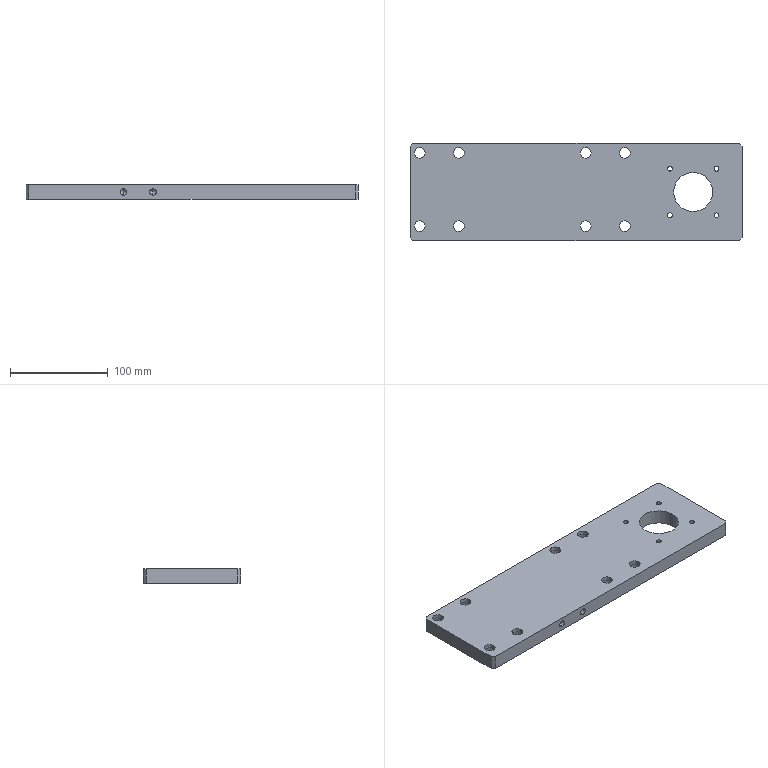Component | SolidWorks | -LowerSlideSleeveConnectionPlate01-1 | 1 solid | 68 faces | box 340 x 100 x 15 mm | volume 465021 mm3 | cylinder 46 | plane 18 | cone 4 | commonest cylinder face diameters 11 x16 17 x16 5 x8 6.8 x4 40 x2
build123d program:
from build123d import *

# Parameters (mm, degrees)
SKETCH1_W             = 340
SKETCH1_H             = 100
BOSS_EXTRUDE1_DEPTH   = 7.5
LPATTERN1_COUNT       = 2
LPATTERN1_PITCH       = 40
LPATTERN1_COUNT_DIR2  = 2
LPATTERN1_PITCH_DIR2  = 75
LPATTERN2_COUNT       = 2
LPATTERN2_PITCH       = 40
LPATTERN2_COUNT_DIR2  = 2
LPATTERN2_PITCH_DIR2  = 75
SKETCH6_R             = 20
CUT_EXTRUDE1_DEPTH    = 15
CIRPATTERN1_COUNT     = 4
CHAMFER1_SIZE         = 3
M8_TAPPED_HOLE1_D     = 6.8
M8_TAPPED_HOLE1_DEPTH = 22.25
M8_TAPPED_HOLE1_TIP   = 2.043


with BuildPart() as part:
    # Sketch1 → Boss-Extrude1 (new, symmetric)
    with BuildSketch(Plane.XY):
        Rectangle(SKETCH1_W, SKETCH1_H)
    extrude(amount=BOSS_EXTRUDE1_DEPTH, both=True)

    # Sketch2 → Cylindrical Countersunk Hole for M10 Hex (revolve, cut)
    with BuildSketch(Plane(origin=(-120, 40, -7.5), x_dir=(0, 1, 0), z_dir=(1, 0, 0))):
        Polygon((0, 0), (0, 25.555), (5.5, 22.25), (5.5, 11), (8.5, 11), (8.5, 0), align=None)
    cylindrical_countersunk_hole_for_m10_hex = revolve(axis=Axis((-120, 40, -13.85), (0, 0, 1)), mode=Mode.SUBTRACT)

    # LPattern1: Cylindrical Countersunk Hole for M10 Hex 2 × 2
    with Locations(*[(-i * LPATTERN1_PITCH, -j * LPATTERN1_PITCH_DIR2, 0) for i in range(LPATTERN1_COUNT) for j in range(LPATTERN1_COUNT_DIR2) if (i, j) != (0, 0)]):
        add(cylindrical_countersunk_hole_for_m10_hex, mode=Mode.SUBTRACT)

    # Sketch4 → Cylindrical Countersunk Hole for M10 2 (revolve, cut)
    with BuildSketch(Plane(origin=(50, 40, -7.5), x_dir=(0, 1, 0), z_dir=(1, 0, 0))):
        Polygon((0, 0), (0, 25.555), (5.5, 22.25), (5.5, 11), (8.5, 11), (8.5, 0), align=None)
    cylindrical_countersunk_hole_for_m10_2 = revolve(axis=Axis((50, 40, -13.85), (0, 0, 1)), mode=Mode.SUBTRACT)

    # LPattern2: Cylindrical Countersunk Hole for M10 2 2 × 2
    with Locations(*[(-i * LPATTERN2_PITCH, -j * LPATTERN2_PITCH_DIR2, 0) for i in range(LPATTERN2_COUNT) for j in range(LPATTERN2_COUNT_DIR2) if (i, j) != (0, 0)]):
        add(cylindrical_countersunk_hole_for_m10_2, mode=Mode.SUBTRACT)

    # Sketch6 → Cut-Extrude1 (cut)
    with BuildSketch(Plane.XY.offset(7.5)):
        with Locations((120, 0)):
            Circle(SKETCH6_R)
    extrude(amount=-CUT_EXTRUDE1_DEPTH, mode=Mode.SUBTRACT)

    # Sketch7 → M6 Tapped Hole1 (revolve, cut)
    with BuildSketch(Plane(origin=(96.135, 23.865, 7.5), x_dir=(0, -1, 0), z_dir=(1, 0, 0))):
        Polygon((0, 0), (0, 18.502), (2.5, 17), (2.5, 0), align=None)
    m6_tapped_hole1 = revolve(axis=Axis((96.135, 23.865, 13.85), (0, 0, -1)), mode=Mode.SUBTRACT)

    # CirPattern1: M6 Tapped Hole1 ×4 about axis
    cirpattern1_axis = Axis((120, 0, 0), (0, 0, 1))
    for i in range(1, CIRPATTERN1_COUNT):
        add(m6_tapped_hole1.rotate(cirpattern1_axis, i * 360 / CIRPATTERN1_COUNT), mode=Mode.SUBTRACT)

    # Chamfer1
    chamfer1_edges = [part.edges().sort_by_distance(p)[0] for p in [
        (170, -50, 0),
        (-170, -50, 0),
        (-170, 50, 0),
        (170, 50, 0),
    ]]
    chamfer(chamfer1_edges, length=CHAMFER1_SIZE)

    # M8 Tapped Hole1
    with Locations(Plane.XZ.offset(50)):
        with Locations((-70, 0), (-40, 0)):
            Hole(M8_TAPPED_HOLE1_D / 2, depth=M8_TAPPED_HOLE1_DEPTH)
            with Locations((0, 0, -(M8_TAPPED_HOLE1_DEPTH + M8_TAPPED_HOLE1_TIP / 2))):  # 118° drill point
                Cone(0, M8_TAPPED_HOLE1_D / 2, M8_TAPPED_HOLE1_TIP, mode=Mode.SUBTRACT)


solid = part.part

# Placed as in the assembly
solid = solid.moved(Location((85, 1094.5, -77.5), (0, 0, 0)))